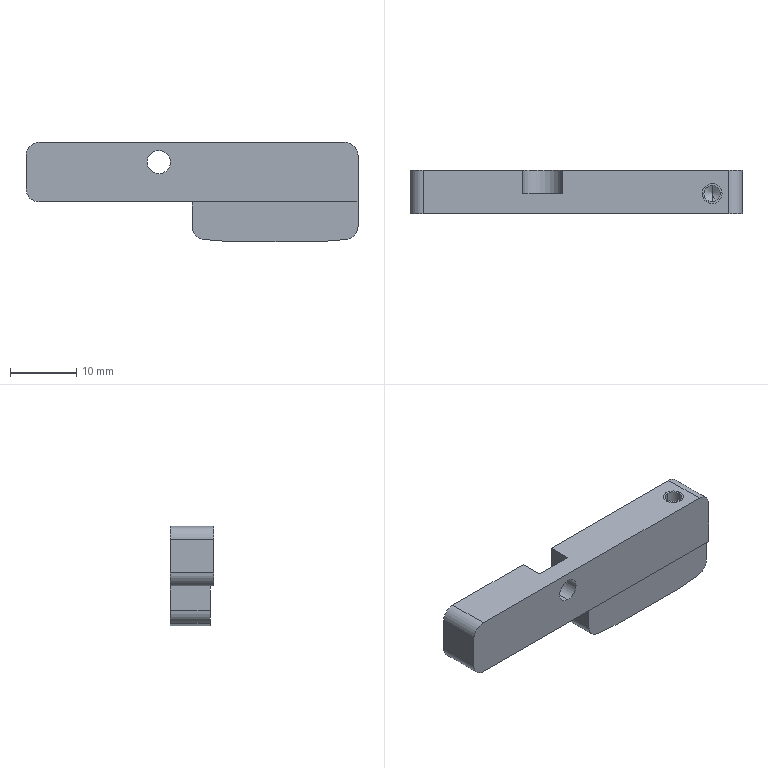CAM job | Mastercam | mm | 1 operations | part box 50 x 6.5 x 15
1. Surface Finish Flowline | 21 - 10 圆鼻铣刀